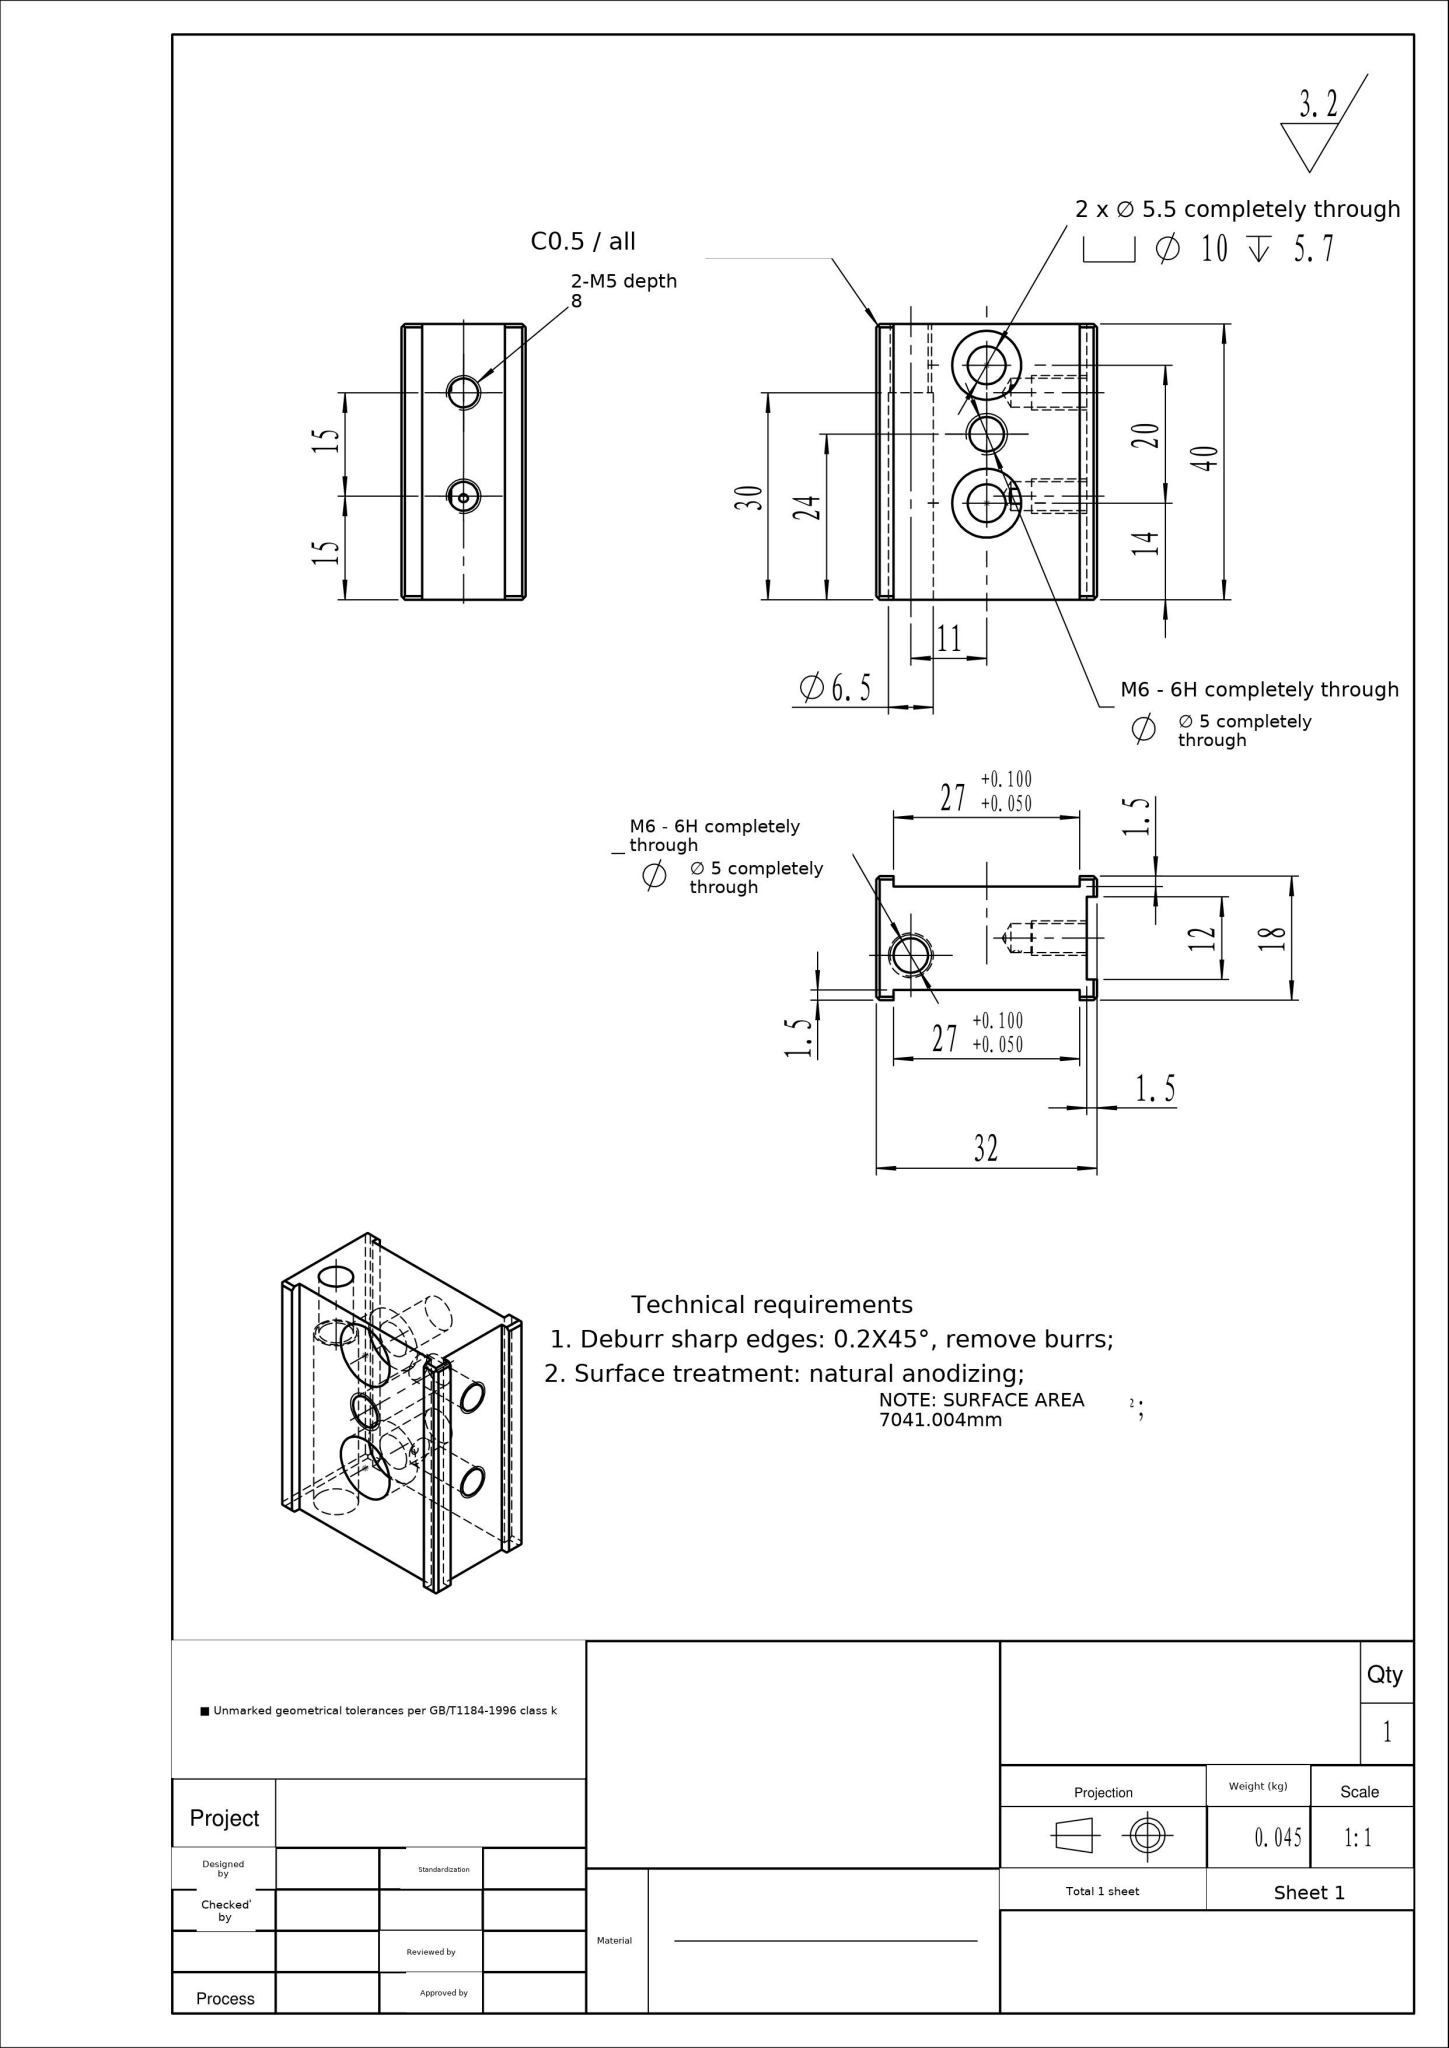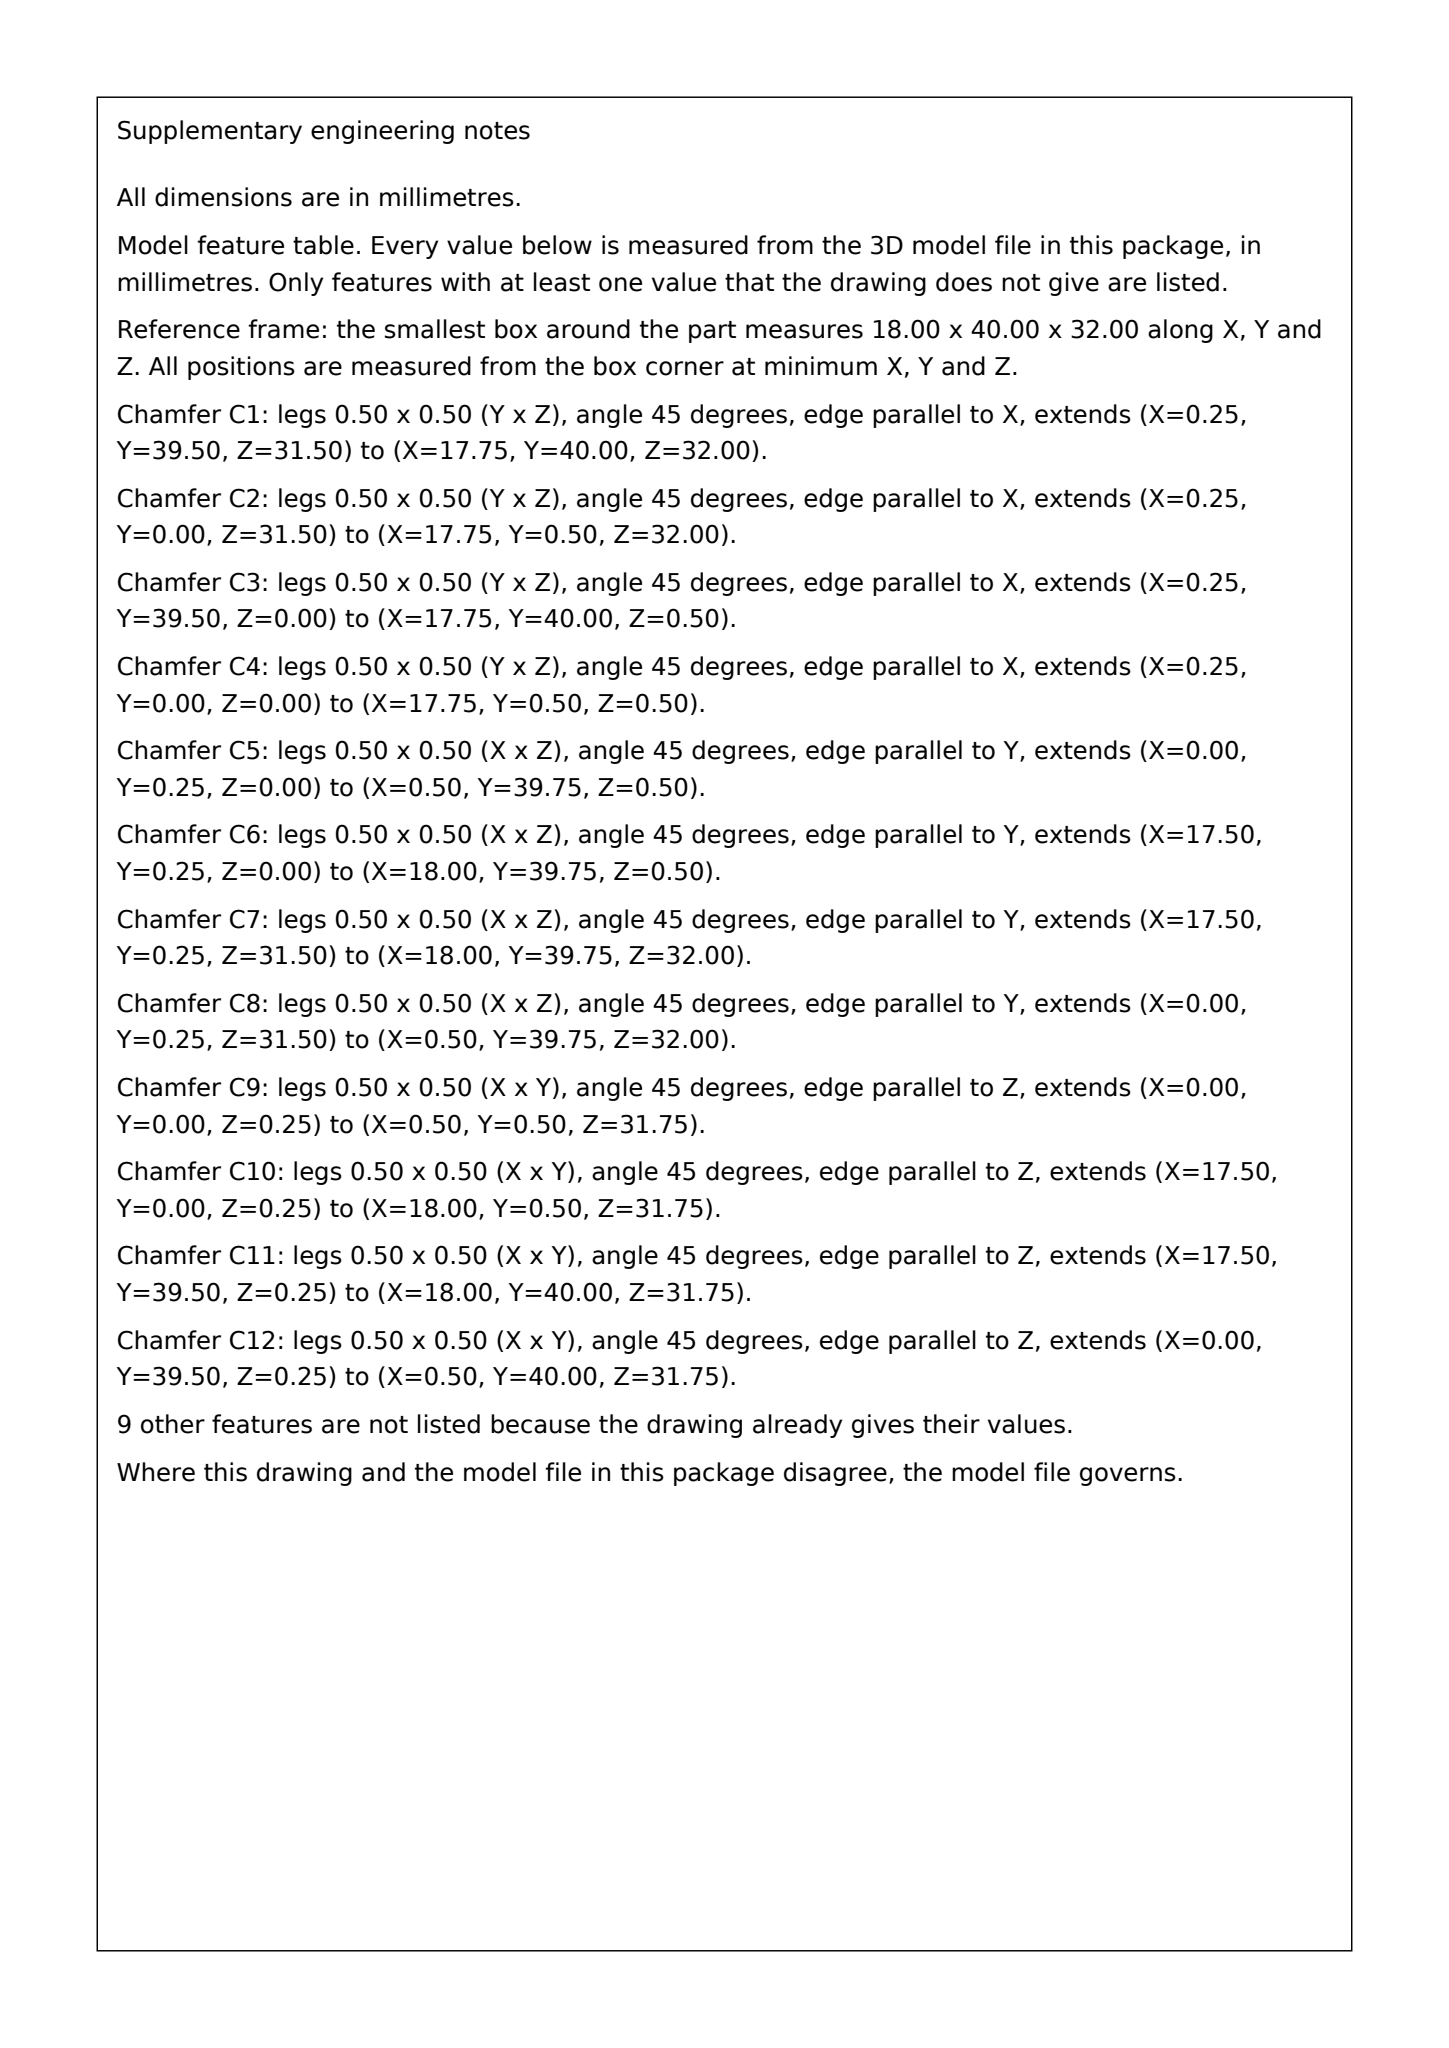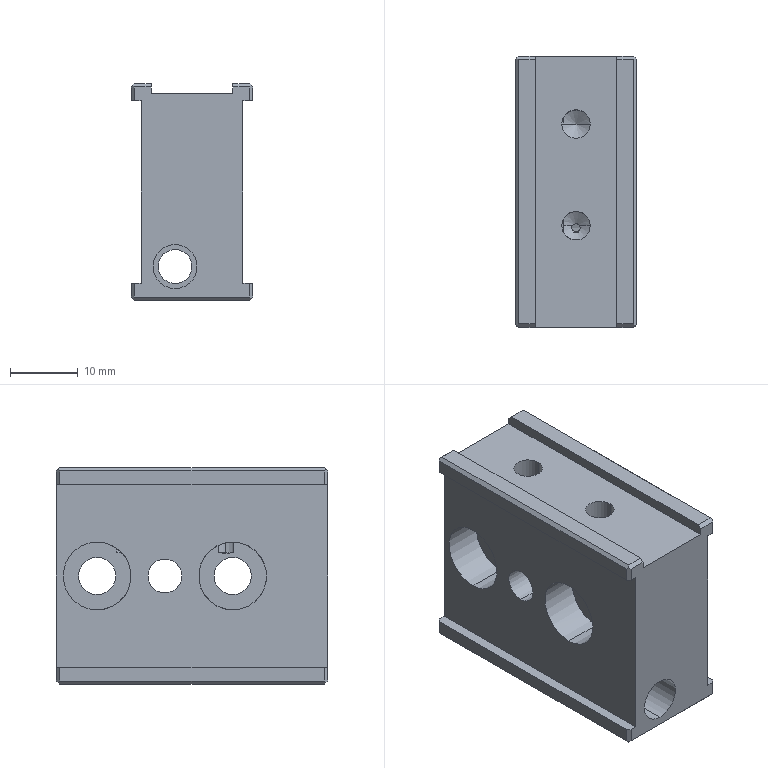Part | SolidWorks | mm | 1 solid | 61 faces | box 18 x 40 x 32 mm | volume 15913 mm3 | plane 39 | cylinder 18 | cone 4 | commonest cylinder face diameters 4.2 x4 5 x4 10 x4 5.5 x4 6.5 x2
build123d program:
from build123d import *

# Parameters (mm, degrees)
SKETCH1_W                                            = 18
SKETCH1_H                                            = 32
BOSS_EXTRUDE1_DEPTH                                  = 40
SKETCH2_W                                            = 1.5
SKETCH2_H                                            = 27
CUT_EXTRUDE1_DEPTH                                   = 45.011
SKETCH6_R                                            = 3.25
CUT_EXTRUDE2_DEPTH                                   = 30
M6_TAPPED_HOLE1_D                                    = 5
CHAMFER2_SIZE                                        = 0.5
CHAMFER3_SIZE                                        = 0.5
HOLE_SIZE_ACCORDING_TO_THE_TYPE_OF_HEXAG_D           = 5.5
HOLE_SIZE_ACCORDING_TO_THE_TYPE_OF_HEXAG_CBORE_D     = 10
HOLE_SIZE_ACCORDING_TO_THE_TYPE_OF_HEXAG_CBORE_DEPTH = 5.7
M6_TAPPED_HOLE2_D                                    = 5
CHAMFER4_SIZE                                        = 0.5
SKETCH15_W                                           = 12
SKETCH15_H                                           = 1.5
CUT_EXTRUDE3_DEPTH                                   = 45.011
M5_TAPPED_HOLE1_D                                    = 4.2
M5_TAPPED_HOLE1_DEPTH                                = 11
M5_TAPPED_HOLE1_TIP                                  = 1.262


with BuildPart() as part:
    # Sketch1 → Boss-Extrude1 (new body)
    with BuildSketch(Plane(origin=(0, 0, 0), x_dir=(1, 0, 0), z_dir=(0, 1, 0))):
        Rectangle(SKETCH1_W, SKETCH1_H)
    extrude(amount=BOSS_EXTRUDE1_DEPTH)

    # Sketch2 → Cut-Extrude1 (cut, through all)
    with BuildSketch(Plane(origin=(0, 40, 0), x_dir=(1, 0, 0), z_dir=(0, 1, 0))):
        with Locations((8.25, 0)):
            Rectangle(SKETCH2_W, SKETCH2_H)
    cut_extrude1 = extrude(amount=-CUT_EXTRUDE1_DEPTH, mode=Mode.SUBTRACT)

    # Sketch6 → Cut-Extrude2 (cut)
    with BuildSketch(Plane.XZ):
        with Locations(Location((-2.5, -11, 0), (0, 0, 270))):
            Circle(SKETCH6_R)
    extrude(amount=-CUT_EXTRUDE2_DEPTH, mode=Mode.SUBTRACT)

    # M6 Tapped Hole1 (through all)
    with Locations(Plane(origin=(0, 30, 0), x_dir=(-1, 0, 0), z_dir=(0, -1, 0))):
        with Locations((2.5, 11)):
            Hole(M6_TAPPED_HOLE1_D / 2)

    # Chamfer2
    chamfer2_edges = [part.edges().sort_by_distance(p)[0] for p in [
        (0, 40, 16),
        (0, 0, 16),
        (0, 0, -16),
        (0, 40, -16),
        (9, 20, 16),
        (-9, 20, 16),
        (-9, 20, -16),
        (9, 20, -16),
    ]]
    chamfer(chamfer2_edges, length=CHAMFER2_SIZE)

    # Chamfer3
    chamfer3_edges = [part.edges().sort_by_distance(p)[0] for p in [
        (9, 0, -14.5),
        (9, 40, -14.5),
        (9, 40, 14.5),
        (-9, 0, 0),
        (9, 0, 14.5),
    ]]
    chamfer(chamfer3_edges, length=CHAMFER3_SIZE)

    # Mirror1: Cut-Extrude1 across plane
    add(cut_extrude1.mirror(Plane(origin=(0, 0, 0), x_dir=(0, 0, 1), z_dir=(1, 0, 0))), mode=Mode.SUBTRACT)

    # Hole Size according to the type of Hexag (through all)
    with Locations(Plane.ZY.offset(7.5)):
        with Locations((0, 14), (0, 34)):
            CounterBoreHole(HOLE_SIZE_ACCORDING_TO_THE_TYPE_OF_HEXAG_D / 2, HOLE_SIZE_ACCORDING_TO_THE_TYPE_OF_HEXAG_CBORE_D / 2, HOLE_SIZE_ACCORDING_TO_THE_TYPE_OF_HEXAG_CBORE_DEPTH)

    # M6 Tapped Hole2 (through all)
    with Locations(Plane.ZY.offset(7.5)):
        with Locations((0, 24)):
            Hole(M6_TAPPED_HOLE2_D / 2)

    # Chamfer4
    chamfer4_edges = [part.edges().sort_by_distance(p)[0] for p in [
        (-9, 40, 14.5),
        (-9, 40, -14.5),
    ]]
    chamfer(chamfer4_edges, length=CHAMFER4_SIZE)

    # Sketch15 → Cut-Extrude3 (cut, through all)
    with BuildSketch(Plane(origin=(0, 40, 0), x_dir=(1, 0, 0), z_dir=(0, 1, 0))):
        with Locations((0, -15.25)):
            Rectangle(SKETCH15_W, SKETCH15_H)
    extrude(amount=-CUT_EXTRUDE3_DEPTH, mode=Mode.SUBTRACT)

    # M5 Tapped Hole1
    with Locations(Plane.XY.offset(14.5)):
        with Locations((0, 30), (0, 15)):
            Hole(M5_TAPPED_HOLE1_D / 2, depth=M5_TAPPED_HOLE1_DEPTH)
            with Locations((0, 0, -(M5_TAPPED_HOLE1_DEPTH + M5_TAPPED_HOLE1_TIP / 2))):  # 118° drill point
                Cone(0, M5_TAPPED_HOLE1_D / 2, M5_TAPPED_HOLE1_TIP, mode=Mode.SUBTRACT)


solid = part.part